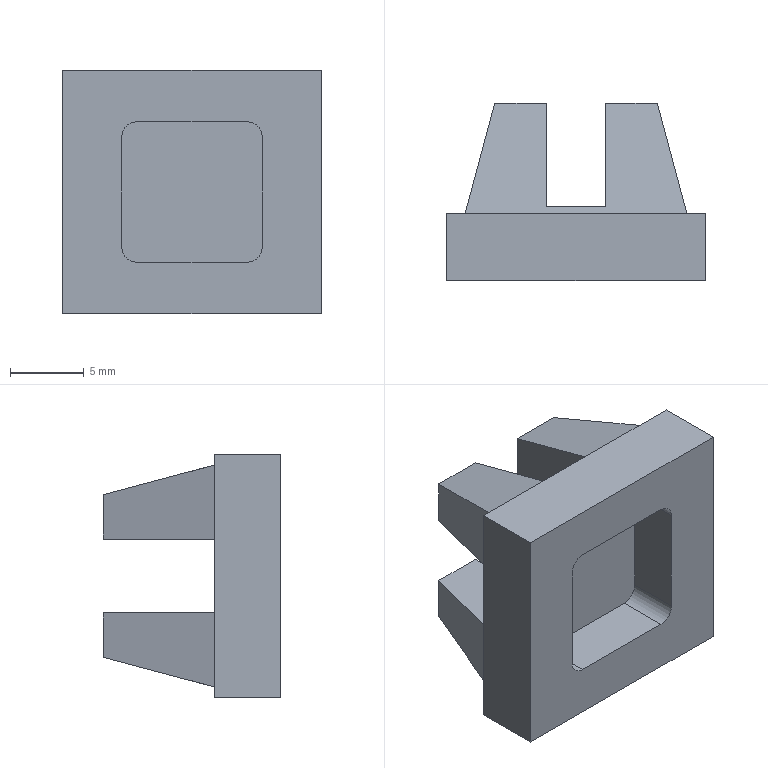Component | NX | SLIDER | 1 solid | 33 faces | volume 1556 mm3 | plane 29 | cylinder 4 | commonest cylinder face diameters 2 x4